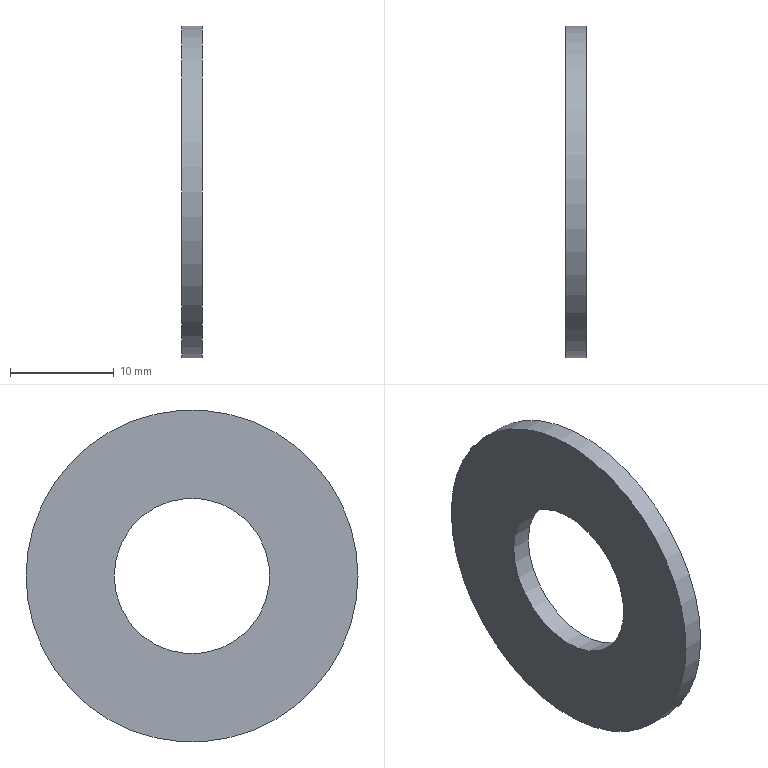Component | NX | WASHER_6 | 1 solid | 4 faces | box 2 x 32 x 32 mm | volume 1255 mm3 | cylinder 2 | plane 2 | commonest cylinder face diameters 32 x1 15 x1
STEP:
#1=CARTESIAN_POINT('',(0.,0.,0.));
#2=DIRECTION('',(0.,0.,1.));
#3=DIRECTION('',(1.,0.,0.));
#4=AXIS2_PLACEMENT_3D('',#1,#2,#3);
#5=CARTESIAN_POINT('',(194.,16.,102.5));
#6=VERTEX_POINT('',#5);
#7=CARTESIAN_POINT('',(194.,0.,102.5));
#8=DIRECTION('',(1.,0.,0.));
#9=DIRECTION('',(0.,1.,0.));
#10=AXIS2_PLACEMENT_3D('',#7,#8,#9);
#11=CIRCLE('',#10,16.);
#12=CARTESIAN_POINT('',(194.,0.,102.5));
#13=DIRECTION('',(-1.,0.,0.));
#14=DIRECTION('',(0.,0.,1.));
#15=AXIS2_PLACEMENT_3D('',#12,#13,#14);
#16=CYLINDRICAL_SURFACE('',#15,16.);
#17=CARTESIAN_POINT('',(7.854,0.));
#18=DIRECTION('',(-1.,0.));
#19=VECTOR('',#18,1.);
#20=LINE('',#17,#19);
#21=(GEOMETRIC_REPRESENTATION_CONTEXT(2)PARAMETRIC_REPRESENTATION_CONTEXT()REPRESENTATION_CONTEXT('',''));
#22=DEFINITIONAL_REPRESENTATION('',(#20),#21);
#23=PCURVE('',#16,#22);
#24=CARTESIAN_POINT('',(194.,0.,102.5));
#25=DIRECTION('',(1.,0.,0.));
#26=DIRECTION('',(0.,0.,-1.));
#27=AXIS2_PLACEMENT_3D('',#24,#25,#26);
#28=PLANE('',#27);
#29=CARTESIAN_POINT('',(0.,0.));
#30=DIRECTION('',(0.,1.));
#31=AXIS2_PLACEMENT_2D('',#29,#30);
#32=CIRCLE('',#31,16.);
#33=(GEOMETRIC_REPRESENTATION_CONTEXT(2)PARAMETRIC_REPRESENTATION_CONTEXT()REPRESENTATION_CONTEXT('',''));
#34=DEFINITIONAL_REPRESENTATION('',(#32),#33);
#35=PCURVE('',#28,#34);
#36=SURFACE_CURVE('',#11,(#23,#35),.PCURVE_S1.);
#37=EDGE_CURVE('',#6,#6,#36,.T.);
#38=ORIENTED_EDGE('',*,*,#37,.F.);
#39=CARTESIAN_POINT('',(192.,16.,102.5));
#40=VERTEX_POINT('',#39);
#41=CARTESIAN_POINT('',(194.,16.,102.5));
#42=CARTESIAN_POINT('',(192.,16.,102.5));
#43=B_SPLINE_CURVE_WITH_KNOTS('',1,(#41,#42),.UNSPECIFIED.,.F.,.F.,(2,2),(0.,2.),.PIECEWISE_BEZIER_KNOTS.);
#44=CARTESIAN_POINT('',(7.854,0.));
#45=DIRECTION('',(0.,1.));
#46=VECTOR('',#45,1.);
#47=LINE('',#44,#46);
#48=(GEOMETRIC_REPRESENTATION_CONTEXT(2)PARAMETRIC_REPRESENTATION_CONTEXT()REPRESENTATION_CONTEXT('',''));
#49=DEFINITIONAL_REPRESENTATION('',(#47),#48);
#50=PCURVE('',#16,#49);
#51=CARTESIAN_POINT('',(1.571,0.));
#52=DIRECTION('',(0.,1.));
#53=VECTOR('',#52,1.);
#54=LINE('',#51,#53);
#55=(GEOMETRIC_REPRESENTATION_CONTEXT(2)PARAMETRIC_REPRESENTATION_CONTEXT()REPRESENTATION_CONTEXT('',''));
#56=DEFINITIONAL_REPRESENTATION('',(#54),#55);
#57=PCURVE('',#16,#56);
#58=SEAM_CURVE('',#43,(#50,#57),.PCURVE_S1.);
#59=EDGE_CURVE('',#6,#40,#58,.T.);
#60=ORIENTED_EDGE('',*,*,#59,.T.);
#61=CARTESIAN_POINT('',(192.,0.,102.5));
#62=DIRECTION('',(1.,0.,0.));
#63=DIRECTION('',(0.,1.,0.));
#64=AXIS2_PLACEMENT_3D('',#61,#62,#63);
#65=CIRCLE('',#64,16.);
#66=CARTESIAN_POINT('',(7.854,2.));
#67=DIRECTION('',(-1.,0.));
#68=VECTOR('',#67,1.);
#69=LINE('',#66,#68);
#70=(GEOMETRIC_REPRESENTATION_CONTEXT(2)PARAMETRIC_REPRESENTATION_CONTEXT()REPRESENTATION_CONTEXT('',''));
#71=DEFINITIONAL_REPRESENTATION('',(#69),#70);
#72=PCURVE('',#16,#71);
#73=CARTESIAN_POINT('',(192.,0.,102.5));
#74=DIRECTION('',(1.,0.,0.));
#75=DIRECTION('',(0.,0.,-1.));
#76=AXIS2_PLACEMENT_3D('',#73,#74,#75);
#77=PLANE('',#76);
#78=CARTESIAN_POINT('',(0.,0.));
#79=DIRECTION('',(0.,1.));
#80=AXIS2_PLACEMENT_2D('',#78,#79);
#81=CIRCLE('',#80,16.);
#82=(GEOMETRIC_REPRESENTATION_CONTEXT(2)PARAMETRIC_REPRESENTATION_CONTEXT()REPRESENTATION_CONTEXT('',''));
#83=DEFINITIONAL_REPRESENTATION('',(#81),#82);
#84=PCURVE('',#77,#83);
#85=SURFACE_CURVE('',#65,(#72,#84),.PCURVE_S1.);
#86=EDGE_CURVE('',#40,#40,#85,.T.);
#87=ORIENTED_EDGE('',*,*,#86,.T.);
#88=ORIENTED_EDGE('',*,*,#59,.F.);
#89=EDGE_LOOP('',(#38,#60,#87,#88));
#90=FACE_BOUND('',#89,.T.);
#91=ADVANCED_FACE('',(#90),#16,.T.);
#92=CARTESIAN_POINT('',(194.,7.5,102.5));
#93=VERTEX_POINT('',#92);
#94=CARTESIAN_POINT('',(194.,0.,102.5));
#95=DIRECTION('',(1.,0.,0.));
#96=DIRECTION('',(0.,1.,0.));
#97=AXIS2_PLACEMENT_3D('',#94,#95,#96);
#98=CIRCLE('',#97,7.5);
#99=CARTESIAN_POINT('',(194.,0.,102.5));
#100=DIRECTION('',(-1.,0.,0.));
#101=DIRECTION('',(0.,0.,1.));
#102=AXIS2_PLACEMENT_3D('',#99,#100,#101);
#103=CYLINDRICAL_SURFACE('',#102,7.5);
#104=CARTESIAN_POINT('',(7.854,0.));
#105=DIRECTION('',(-1.,0.));
#106=VECTOR('',#105,1.);
#107=LINE('',#104,#106);
#108=(GEOMETRIC_REPRESENTATION_CONTEXT(2)PARAMETRIC_REPRESENTATION_CONTEXT()REPRESENTATION_CONTEXT('',''));
#109=DEFINITIONAL_REPRESENTATION('',(#107),#108);
#110=PCURVE('',#103,#109);
#111=CARTESIAN_POINT('',(0.,0.));
#112=DIRECTION('',(0.,1.));
#113=AXIS2_PLACEMENT_2D('',#111,#112);
#114=CIRCLE('',#113,7.5);
#115=(GEOMETRIC_REPRESENTATION_CONTEXT(2)PARAMETRIC_REPRESENTATION_CONTEXT()REPRESENTATION_CONTEXT('',''));
#116=DEFINITIONAL_REPRESENTATION('',(#114),#115);
#117=PCURVE('',#28,#116);
#118=SURFACE_CURVE('',#98,(#110,#117),.PCURVE_S1.);
#119=EDGE_CURVE('',#93,#93,#118,.T.);
#120=ORIENTED_EDGE('',*,*,#119,.F.);
#121=CARTESIAN_POINT('',(192.,7.5,102.5));
#122=VERTEX_POINT('',#121);
#123=CARTESIAN_POINT('',(194.,7.5,102.5));
#124=CARTESIAN_POINT('',(192.,7.5,102.5));
#125=B_SPLINE_CURVE_WITH_KNOTS('',1,(#123,#124),.UNSPECIFIED.,.F.,.F.,(2,2),(0.,2.),.PIECEWISE_BEZIER_KNOTS.);
#126=CARTESIAN_POINT('',(7.854,0.));
#127=DIRECTION('',(0.,1.));
#128=VECTOR('',#127,1.);
#129=LINE('',#126,#128);
#130=(GEOMETRIC_REPRESENTATION_CONTEXT(2)PARAMETRIC_REPRESENTATION_CONTEXT()REPRESENTATION_CONTEXT('',''));
#131=DEFINITIONAL_REPRESENTATION('',(#129),#130);
#132=PCURVE('',#103,#131);
#133=CARTESIAN_POINT('',(1.571,0.));
#134=DIRECTION('',(0.,1.));
#135=VECTOR('',#134,1.);
#136=LINE('',#133,#135);
#137=(GEOMETRIC_REPRESENTATION_CONTEXT(2)PARAMETRIC_REPRESENTATION_CONTEXT()REPRESENTATION_CONTEXT('',''));
#138=DEFINITIONAL_REPRESENTATION('',(#136),#137);
#139=PCURVE('',#103,#138);
#140=SEAM_CURVE('',#125,(#132,#139),.PCURVE_S1.);
#141=EDGE_CURVE('',#93,#122,#140,.T.);
#142=ORIENTED_EDGE('',*,*,#141,.T.);
#143=CARTESIAN_POINT('',(192.,0.,102.5));
#144=DIRECTION('',(1.,0.,0.));
#145=DIRECTION('',(0.,1.,0.));
#146=AXIS2_PLACEMENT_3D('',#143,#144,#145);
#147=CIRCLE('',#146,7.5);
#148=CARTESIAN_POINT('',(7.854,2.));
#149=DIRECTION('',(-1.,0.));
#150=VECTOR('',#149,1.);
#151=LINE('',#148,#150);
#152=(GEOMETRIC_REPRESENTATION_CONTEXT(2)PARAMETRIC_REPRESENTATION_CONTEXT()REPRESENTATION_CONTEXT('',''));
#153=DEFINITIONAL_REPRESENTATION('',(#151),#152);
#154=PCURVE('',#103,#153);
#155=CARTESIAN_POINT('',(0.,0.));
#156=DIRECTION('',(0.,1.));
#157=AXIS2_PLACEMENT_2D('',#155,#156);
#158=CIRCLE('',#157,7.5);
#159=(GEOMETRIC_REPRESENTATION_CONTEXT(2)PARAMETRIC_REPRESENTATION_CONTEXT()REPRESENTATION_CONTEXT('',''));
#160=DEFINITIONAL_REPRESENTATION('',(#158),#159);
#161=PCURVE('',#77,#160);
#162=SURFACE_CURVE('',#147,(#154,#161),.PCURVE_S1.);
#163=EDGE_CURVE('',#122,#122,#162,.T.);
#164=ORIENTED_EDGE('',*,*,#163,.T.);
#165=ORIENTED_EDGE('',*,*,#141,.F.);
#166=EDGE_LOOP('',(#120,#142,#164,#165));
#167=FACE_BOUND('',#166,.F.);
#168=ADVANCED_FACE('',(#167),#103,.F.);
#169=ORIENTED_EDGE('',*,*,#37,.T.);
#170=EDGE_LOOP('',(#169));
#171=FACE_BOUND('',#170,.T.);
#172=ORIENTED_EDGE('',*,*,#119,.F.);
#173=EDGE_LOOP('',(#172));
#174=FACE_BOUND('',#173,.T.);
#175=ADVANCED_FACE('',(#171,#174),#28,.T.);
#176=ORIENTED_EDGE('',*,*,#86,.F.);
#177=EDGE_LOOP('',(#176));
#178=FACE_BOUND('',#177,.T.);
#179=ORIENTED_EDGE('',*,*,#163,.T.);
#180=EDGE_LOOP('',(#179));
#181=FACE_BOUND('',#180,.T.);
#182=ADVANCED_FACE('',(#178,#181),#77,.F.);
#183=CLOSED_SHELL('',(#91,#168,#175,#182));
#184=MANIFOLD_SOLID_BREP('',#183);
#185=(LENGTH_UNIT()NAMED_UNIT(*)SI_UNIT(.MILLI.,.METRE.));
#186=UNCERTAINTY_MEASURE_WITH_UNIT(LENGTH_MEASURE(0.00001),#185,'','');
#187=(NAMED_UNIT(*)PLANE_ANGLE_UNIT()SI_UNIT($,.RADIAN.));
#188=(NAMED_UNIT(*)SI_UNIT($,.STERADIAN.)SOLID_ANGLE_UNIT());
#189=(GEOMETRIC_REPRESENTATION_CONTEXT(3)GLOBAL_UNCERTAINTY_ASSIGNED_CONTEXT((#186))GLOBAL_UNIT_ASSIGNED_CONTEXT((#185,#187,#188))REPRESENTATION_CONTEXT('',''));
#190=ADVANCED_BREP_SHAPE_REPRESENTATION('',(#4,#184),#189);